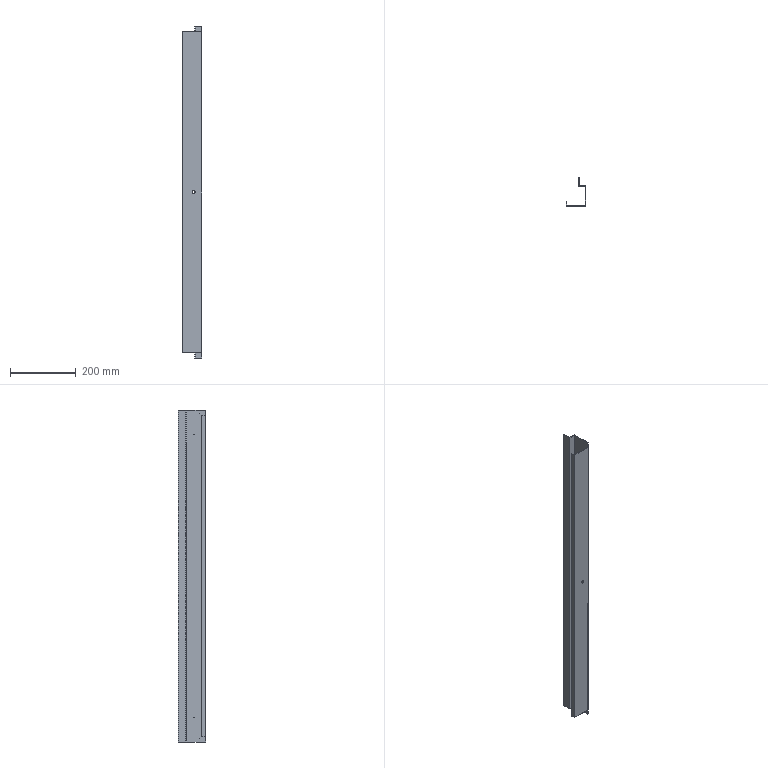Component | SolidWorks | CabinetWelding-1_RearLowerBeam-1 | 1 solid | 60 faces | volume 207073 mm3 | plane 30 | cylinder 28 | spline 2 | commonest cylinder face diameters 0.5 x8 5.2 x6 3 x4 0.4 x4 2.8 x4 8.5 x2